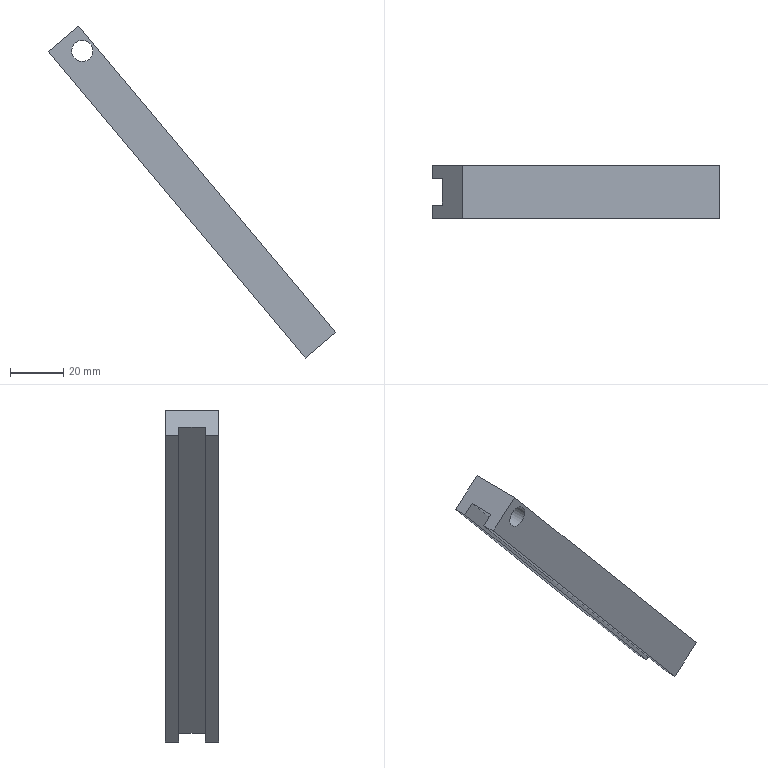Component | NX | MODEL7 | 1 solid | 11 faces | box 107.91 x 20 x 124.55 mm | volume 36495 mm3 | plane 10 | cylinder 1 | commonest cylinder face diameters 8 x1
STEP:
#1=CARTESIAN_POINT('',(0.,0.,0.));
#2=DIRECTION('',(0.,0.,1.));
#3=DIRECTION('',(1.,0.,0.));
#4=AXIS2_PLACEMENT_3D('',#1,#2,#3);
#5=CARTESIAN_POINT('',(827.663,10.431,-119.455));
#6=VERTEX_POINT('',#5);
#7=CARTESIAN_POINT('',(924.081,10.431,-234.362));
#8=VERTEX_POINT('',#7);
#9=CARTESIAN_POINT('',(827.663,10.431,-119.455));
#10=DIRECTION('',(0.6428,0.,-0.766));
#11=VECTOR('',#10,1.);
#12=LINE('',#9,#11);
#13=CARTESIAN_POINT('',(827.663,-4.569,-119.455));
#14=DIRECTION('',(0.766,0.,0.6428));
#15=DIRECTION('',(0.,-1.,0.));
#16=AXIS2_PLACEMENT_3D('',#13,#14,#15);
#17=PLANE('',#16);
#18=CARTESIAN_POINT('',(-15.,0.));
#19=DIRECTION('',(0.,1.));
#20=VECTOR('',#19,1.);
#21=LINE('',#18,#20);
#22=(GEOMETRIC_REPRESENTATION_CONTEXT(2)PARAMETRIC_REPRESENTATION_CONTEXT()REPRESENTATION_CONTEXT('',''));
#23=DEFINITIONAL_REPRESENTATION('',(#21),#22);
#24=PCURVE('',#17,#23);
#25=CARTESIAN_POINT('',(831.493,10.431,-116.241));
#26=DIRECTION('',(0.,1.,0.));
#27=DIRECTION('',(-0.6428,0.,0.766));
#28=AXIS2_PLACEMENT_3D('',#25,#26,#27);
#29=PLANE('',#28);
#30=CARTESIAN_POINT('',(0.,-5.));
#31=DIRECTION('',(-1.,0.));
#32=VECTOR('',#31,1.);
#33=LINE('',#30,#32);
#34=(GEOMETRIC_REPRESENTATION_CONTEXT(2)PARAMETRIC_REPRESENTATION_CONTEXT()REPRESENTATION_CONTEXT('',''));
#35=DEFINITIONAL_REPRESENTATION('',(#33),#34);
#36=PCURVE('',#29,#35);
#37=SURFACE_CURVE('',#12,(#24,#36),.PCURVE_S1.);
#38=EDGE_CURVE('',#6,#8,#37,.T.);
#39=ORIENTED_EDGE('',*,*,#38,.F.);
#40=CARTESIAN_POINT('',(827.663,15.431,-119.455));
#41=VERTEX_POINT('',#40);
#42=CARTESIAN_POINT('',(827.663,-4.569,-119.455));
#43=DIRECTION('',(0.,1.,0.));
#44=VECTOR('',#43,1.);
#45=LINE('',#42,#44);
#46=CARTESIAN_POINT('',(0.,0.));
#47=DIRECTION('',(-1.,0.));
#48=VECTOR('',#47,1.);
#49=LINE('',#46,#48);
#50=(GEOMETRIC_REPRESENTATION_CONTEXT(2)PARAMETRIC_REPRESENTATION_CONTEXT()REPRESENTATION_CONTEXT('',''));
#51=DEFINITIONAL_REPRESENTATION('',(#49),#50);
#52=PCURVE('',#17,#51);
#53=CARTESIAN_POINT('',(839.154,-4.569,-109.813));
#54=DIRECTION('',(0.6428,0.,-0.766));
#55=DIRECTION('',(0.,1.,0.));
#56=AXIS2_PLACEMENT_3D('',#53,#54,#55);
#57=PLANE('',#56);
#58=CARTESIAN_POINT('',(0.,-15.));
#59=DIRECTION('',(1.,0.));
#60=VECTOR('',#59,1.);
#61=LINE('',#58,#60);
#62=(GEOMETRIC_REPRESENTATION_CONTEXT(2)PARAMETRIC_REPRESENTATION_CONTEXT()REPRESENTATION_CONTEXT('',''));
#63=DEFINITIONAL_REPRESENTATION('',(#61),#62);
#64=PCURVE('',#57,#63);
#65=SURFACE_CURVE('',#45,(#52,#64),.PCURVE_S1.);
#66=EDGE_CURVE('',#6,#41,#65,.T.);
#67=ORIENTED_EDGE('',*,*,#66,.T.);
#68=CARTESIAN_POINT('',(924.081,15.431,-234.362));
#69=VERTEX_POINT('',#68);
#70=CARTESIAN_POINT('',(827.663,15.431,-119.455));
#71=DIRECTION('',(0.6428,0.,-0.766));
#72=VECTOR('',#71,1.);
#73=LINE('',#70,#72);
#74=CARTESIAN_POINT('',(-20.,0.));
#75=DIRECTION('',(0.,1.));
#76=VECTOR('',#75,1.);
#77=LINE('',#74,#76);
#78=(GEOMETRIC_REPRESENTATION_CONTEXT(2)PARAMETRIC_REPRESENTATION_CONTEXT()REPRESENTATION_CONTEXT('',''));
#79=DEFINITIONAL_REPRESENTATION('',(#77),#78);
#80=PCURVE('',#17,#79);
#81=CARTESIAN_POINT('',(827.663,15.431,-119.455));
#82=DIRECTION('',(0.,-1.,0.));
#83=DIRECTION('',(0.6428,0.,-0.766));
#84=AXIS2_PLACEMENT_3D('',#81,#82,#83);
#85=PLANE('',#84);
#86=CARTESIAN_POINT('',(0.,0.));
#87=DIRECTION('',(1.,0.));
#88=VECTOR('',#87,1.);
#89=LINE('',#86,#88);
#90=(GEOMETRIC_REPRESENTATION_CONTEXT(2)PARAMETRIC_REPRESENTATION_CONTEXT()REPRESENTATION_CONTEXT('',''));
#91=DEFINITIONAL_REPRESENTATION('',(#89),#90);
#92=PCURVE('',#85,#91);
#93=SURFACE_CURVE('',#73,(#80,#92),.PCURVE_S1.);
#94=EDGE_CURVE('',#41,#69,#93,.T.);
#95=ORIENTED_EDGE('',*,*,#94,.T.);
#96=CARTESIAN_POINT('',(924.081,-4.569,-234.362));
#97=DIRECTION('',(0.,1.,0.));
#98=VECTOR('',#97,1.);
#99=LINE('',#96,#98);
#100=CARTESIAN_POINT('',(0.,150.));
#101=DIRECTION('',(-1.,0.));
#102=VECTOR('',#101,1.);
#103=LINE('',#100,#102);
#104=(GEOMETRIC_REPRESENTATION_CONTEXT(2)PARAMETRIC_REPRESENTATION_CONTEXT()REPRESENTATION_CONTEXT('',''));
#105=DEFINITIONAL_REPRESENTATION('',(#103),#104);
#106=PCURVE('',#17,#105);
#107=CARTESIAN_POINT('',(924.081,-4.569,-234.362));
#108=DIRECTION('',(-0.6428,0.,0.766));
#109=DIRECTION('',(0.,-1.,0.));
#110=AXIS2_PLACEMENT_3D('',#107,#108,#109);
#111=PLANE('',#110);
#112=CARTESIAN_POINT('',(0.,0.));
#113=DIRECTION('',(-1.,0.));
#114=VECTOR('',#113,1.);
#115=LINE('',#112,#114);
#116=(GEOMETRIC_REPRESENTATION_CONTEXT(2)PARAMETRIC_REPRESENTATION_CONTEXT()REPRESENTATION_CONTEXT('',''));
#117=DEFINITIONAL_REPRESENTATION('',(#115),#116);
#118=PCURVE('',#111,#117);
#119=SURFACE_CURVE('',#99,(#106,#118),.PCURVE_S1.);
#120=EDGE_CURVE('',#8,#69,#119,.T.);
#121=ORIENTED_EDGE('',*,*,#120,.F.);
#122=EDGE_LOOP('',(#39,#67,#95,#121));
#123=FACE_BOUND('',#122,.T.);
#124=ADVANCED_FACE('',(#123),#17,.F.);
#125=CARTESIAN_POINT('',(924.081,0.4306,-234.362));
#126=VERTEX_POINT('',#125);
#127=CARTESIAN_POINT('',(827.663,0.4306,-119.455));
#128=VERTEX_POINT('',#127);
#129=CARTESIAN_POINT('',(924.081,0.4306,-234.362));
#130=DIRECTION('',(-0.6428,0.,0.766));
#131=VECTOR('',#130,1.);
#132=LINE('',#129,#131);
#133=CARTESIAN_POINT('',(827.663,-4.569,-119.455));
#134=DIRECTION('',(0.766,0.,0.6428));
#135=DIRECTION('',(0.,-1.,0.));
#136=AXIS2_PLACEMENT_3D('',#133,#134,#135);
#137=PLANE('',#136);
#138=CARTESIAN_POINT('',(-5.,150.));
#139=DIRECTION('',(0.,-1.));
#140=VECTOR('',#139,1.);
#141=LINE('',#138,#140);
#142=(GEOMETRIC_REPRESENTATION_CONTEXT(2)PARAMETRIC_REPRESENTATION_CONTEXT()REPRESENTATION_CONTEXT('',''));
#143=DEFINITIONAL_REPRESENTATION('',(#141),#142);
#144=PCURVE('',#137,#143);
#145=CARTESIAN_POINT('',(927.911,0.4306,-231.148));
#146=DIRECTION('',(0.,-1.,0.));
#147=DIRECTION('',(0.6428,0.,-0.766));
#148=AXIS2_PLACEMENT_3D('',#145,#146,#147);
#149=PLANE('',#148);
#150=CARTESIAN_POINT('',(0.,-5.));
#151=DIRECTION('',(-1.,0.));
#152=VECTOR('',#151,1.);
#153=LINE('',#150,#152);
#154=(GEOMETRIC_REPRESENTATION_CONTEXT(2)PARAMETRIC_REPRESENTATION_CONTEXT()REPRESENTATION_CONTEXT('',''));
#155=DEFINITIONAL_REPRESENTATION('',(#153),#154);
#156=PCURVE('',#149,#155);
#157=SURFACE_CURVE('',#132,(#144,#156),.PCURVE_S1.);
#158=EDGE_CURVE('',#126,#128,#157,.T.);
#159=ORIENTED_EDGE('',*,*,#158,.F.);
#160=CARTESIAN_POINT('',(924.081,-4.569,-234.362));
#161=VERTEX_POINT('',#160);
#162=CARTESIAN_POINT('',(924.081,-4.569,-234.362));
#163=DIRECTION('',(0.,1.,0.));
#164=VECTOR('',#163,1.);
#165=LINE('',#162,#164);
#166=CARTESIAN_POINT('',(0.,150.));
#167=DIRECTION('',(-1.,0.));
#168=VECTOR('',#167,1.);
#169=LINE('',#166,#168);
#170=(GEOMETRIC_REPRESENTATION_CONTEXT(2)PARAMETRIC_REPRESENTATION_CONTEXT()REPRESENTATION_CONTEXT('',''));
#171=DEFINITIONAL_REPRESENTATION('',(#169),#170);
#172=PCURVE('',#137,#171);
#173=CARTESIAN_POINT('',(0.,0.));
#174=DIRECTION('',(-1.,0.));
#175=VECTOR('',#174,1.);
#176=LINE('',#173,#175);
#177=(GEOMETRIC_REPRESENTATION_CONTEXT(2)PARAMETRIC_REPRESENTATION_CONTEXT()REPRESENTATION_CONTEXT('',''));
#178=DEFINITIONAL_REPRESENTATION('',(#176),#177);
#179=PCURVE('',#111,#178);
#180=SURFACE_CURVE('',#165,(#172,#179),.PCURVE_S1.);
#181=EDGE_CURVE('',#161,#126,#180,.T.);
#182=ORIENTED_EDGE('',*,*,#181,.F.);
#183=CARTESIAN_POINT('',(827.663,-4.569,-119.455));
#184=VERTEX_POINT('',#183);
#185=CARTESIAN_POINT('',(827.663,-4.569,-119.455));
#186=DIRECTION('',(0.6428,0.,-0.766));
#187=VECTOR('',#186,1.);
#188=LINE('',#185,#187);
#189=CARTESIAN_POINT('',(0.,0.));
#190=DIRECTION('',(0.,1.));
#191=VECTOR('',#190,1.);
#192=LINE('',#189,#191);
#193=(GEOMETRIC_REPRESENTATION_CONTEXT(2)PARAMETRIC_REPRESENTATION_CONTEXT()REPRESENTATION_CONTEXT('',''));
#194=DEFINITIONAL_REPRESENTATION('',(#192),#193);
#195=PCURVE('',#137,#194);
#196=CARTESIAN_POINT('',(827.663,-4.569,-119.455));
#197=DIRECTION('',(0.,-1.,0.));
#198=DIRECTION('',(0.6428,0.,-0.766));
#199=AXIS2_PLACEMENT_3D('',#196,#197,#198);
#200=PLANE('',#199);
#201=CARTESIAN_POINT('',(0.,0.));
#202=DIRECTION('',(1.,0.));
#203=VECTOR('',#202,1.);
#204=LINE('',#201,#203);
#205=(GEOMETRIC_REPRESENTATION_CONTEXT(2)PARAMETRIC_REPRESENTATION_CONTEXT()REPRESENTATION_CONTEXT('',''));
#206=DEFINITIONAL_REPRESENTATION('',(#204),#205);
#207=PCURVE('',#200,#206);
#208=SURFACE_CURVE('',#188,(#195,#207),.PCURVE_S1.);
#209=EDGE_CURVE('',#184,#161,#208,.T.);
#210=ORIENTED_EDGE('',*,*,#209,.F.);
#211=CARTESIAN_POINT('',(827.663,-4.569,-119.455));
#212=DIRECTION('',(0.,1.,0.));
#213=VECTOR('',#212,1.);
#214=LINE('',#211,#213);
#215=CARTESIAN_POINT('',(0.,0.));
#216=DIRECTION('',(-1.,0.));
#217=VECTOR('',#216,1.);
#218=LINE('',#215,#217);
#219=(GEOMETRIC_REPRESENTATION_CONTEXT(2)PARAMETRIC_REPRESENTATION_CONTEXT()REPRESENTATION_CONTEXT('',''));
#220=DEFINITIONAL_REPRESENTATION('',(#218),#219);
#221=PCURVE('',#137,#220);
#222=CARTESIAN_POINT('',(0.,-15.));
#223=DIRECTION('',(1.,0.));
#224=VECTOR('',#223,1.);
#225=LINE('',#222,#224);
#226=(GEOMETRIC_REPRESENTATION_CONTEXT(2)PARAMETRIC_REPRESENTATION_CONTEXT()REPRESENTATION_CONTEXT('',''));
#227=DEFINITIONAL_REPRESENTATION('',(#225),#226);
#228=PCURVE('',#57,#227);
#229=SURFACE_CURVE('',#214,(#221,#228),.PCURVE_S1.);
#230=EDGE_CURVE('',#184,#128,#229,.T.);
#231=ORIENTED_EDGE('',*,*,#230,.T.);
#232=EDGE_LOOP('',(#159,#182,#210,#231));
#233=FACE_BOUND('',#232,.T.);
#234=ADVANCED_FACE('',(#233),#137,.F.);
#235=CARTESIAN_POINT('',(831.493,0.4306,-116.241));
#236=VERTEX_POINT('',#235);
#237=CARTESIAN_POINT('',(831.493,10.431,-116.241));
#238=VERTEX_POINT('',#237);
#239=CARTESIAN_POINT('',(831.493,0.4306,-116.241));
#240=DIRECTION('',(0.,1.,0.));
#241=VECTOR('',#240,1.);
#242=LINE('',#239,#241);
#243=CARTESIAN_POINT('',(5.,-10.));
#244=DIRECTION('',(1.,0.));
#245=VECTOR('',#244,1.);
#246=LINE('',#243,#245);
#247=(GEOMETRIC_REPRESENTATION_CONTEXT(2)PARAMETRIC_REPRESENTATION_CONTEXT()REPRESENTATION_CONTEXT('',''));
#248=DEFINITIONAL_REPRESENTATION('',(#246),#247);
#249=PCURVE('',#57,#248);
#250=CARTESIAN_POINT('',(831.493,15.431,-116.241));
#251=DIRECTION('',(-0.766,0.,-0.6428));
#252=DIRECTION('',(0.,1.,0.));
#253=AXIS2_PLACEMENT_3D('',#250,#251,#252);
#254=PLANE('',#253);
#255=CARTESIAN_POINT('',(-15.,0.));
#256=DIRECTION('',(1.,0.));
#257=VECTOR('',#256,1.);
#258=LINE('',#255,#257);
#259=(GEOMETRIC_REPRESENTATION_CONTEXT(2)PARAMETRIC_REPRESENTATION_CONTEXT()REPRESENTATION_CONTEXT('',''));
#260=DEFINITIONAL_REPRESENTATION('',(#258),#259);
#261=PCURVE('',#254,#260);
#262=SURFACE_CURVE('',#242,(#249,#261),.PCURVE_S1.);
#263=EDGE_CURVE('',#236,#238,#262,.T.);
#264=ORIENTED_EDGE('',*,*,#263,.F.);
#265=CARTESIAN_POINT('',(831.493,0.4306,-116.241));
#266=DIRECTION('',(-0.766,0.,-0.6428));
#267=VECTOR('',#266,1.);
#268=LINE('',#265,#267);
#269=CARTESIAN_POINT('',(5.,-10.));
#270=DIRECTION('',(0.,-1.));
#271=VECTOR('',#270,1.);
#272=LINE('',#269,#271);
#273=(GEOMETRIC_REPRESENTATION_CONTEXT(2)PARAMETRIC_REPRESENTATION_CONTEXT()REPRESENTATION_CONTEXT('',''));
#274=DEFINITIONAL_REPRESENTATION('',(#272),#273);
#275=PCURVE('',#57,#274);
#276=CARTESIAN_POINT('',(-150.,-0.));
#277=DIRECTION('',(-0.,-1.));
#278=VECTOR('',#277,1.);
#279=LINE('',#276,#278);
#280=(GEOMETRIC_REPRESENTATION_CONTEXT(2)PARAMETRIC_REPRESENTATION_CONTEXT()REPRESENTATION_CONTEXT('',''));
#281=DEFINITIONAL_REPRESENTATION('',(#279),#280);
#282=PCURVE('',#149,#281);
#283=SURFACE_CURVE('',#268,(#275,#282),.PCURVE_S1.);
#284=EDGE_CURVE('',#236,#128,#283,.T.);
#285=ORIENTED_EDGE('',*,*,#284,.T.);
#286=ORIENTED_EDGE('',*,*,#230,.F.);
#287=CARTESIAN_POINT('',(839.154,-4.569,-109.813));
#288=VERTEX_POINT('',#287);
#289=CARTESIAN_POINT('',(839.154,-4.569,-109.813));
#290=DIRECTION('',(-0.766,0.,-0.6428));
#291=VECTOR('',#290,1.);
#292=LINE('',#289,#291);
#293=CARTESIAN_POINT('',(0.,0.));
#294=DIRECTION('',(0.,-1.));
#295=VECTOR('',#294,1.);
#296=LINE('',#293,#295);
#297=(GEOMETRIC_REPRESENTATION_CONTEXT(2)PARAMETRIC_REPRESENTATION_CONTEXT()REPRESENTATION_CONTEXT('',''));
#298=DEFINITIONAL_REPRESENTATION('',(#296),#297);
#299=PCURVE('',#57,#298);
#300=CARTESIAN_POINT('',(-0.,15.));
#301=DIRECTION('',(0.,-1.));
#302=VECTOR('',#301,1.);
#303=LINE('',#300,#302);
#304=(GEOMETRIC_REPRESENTATION_CONTEXT(2)PARAMETRIC_REPRESENTATION_CONTEXT()REPRESENTATION_CONTEXT('',''));
#305=DEFINITIONAL_REPRESENTATION('',(#303),#304);
#306=PCURVE('',#200,#305);
#307=SURFACE_CURVE('',#292,(#299,#306),.PCURVE_S1.);
#308=EDGE_CURVE('',#288,#184,#307,.T.);
#309=ORIENTED_EDGE('',*,*,#308,.F.);
#310=CARTESIAN_POINT('',(839.154,15.431,-109.813));
#311=VERTEX_POINT('',#310);
#312=CARTESIAN_POINT('',(839.154,-4.569,-109.813));
#313=DIRECTION('',(0.,1.,0.));
#314=VECTOR('',#313,1.);
#315=LINE('',#312,#314);
#316=CARTESIAN_POINT('',(0.,0.));
#317=DIRECTION('',(1.,0.));
#318=VECTOR('',#317,1.);
#319=LINE('',#316,#318);
#320=(GEOMETRIC_REPRESENTATION_CONTEXT(2)PARAMETRIC_REPRESENTATION_CONTEXT()REPRESENTATION_CONTEXT('',''));
#321=DEFINITIONAL_REPRESENTATION('',(#319),#320);
#322=PCURVE('',#57,#321);
#323=CARTESIAN_POINT('',(935.572,-4.569,-224.72));
#324=DIRECTION('',(-0.766,0.,-0.6428));
#325=DIRECTION('',(0.,1.,0.));
#326=AXIS2_PLACEMENT_3D('',#323,#324,#325);
#327=PLANE('',#326);
#328=CARTESIAN_POINT('',(0.,-150.));
#329=DIRECTION('',(1.,0.));
#330=VECTOR('',#329,1.);
#331=LINE('',#328,#330);
#332=(GEOMETRIC_REPRESENTATION_CONTEXT(2)PARAMETRIC_REPRESENTATION_CONTEXT()REPRESENTATION_CONTEXT('',''));
#333=DEFINITIONAL_REPRESENTATION('',(#331),#332);
#334=PCURVE('',#327,#333);
#335=SURFACE_CURVE('',#315,(#322,#334),.PCURVE_S1.);
#336=EDGE_CURVE('',#288,#311,#335,.T.);
#337=ORIENTED_EDGE('',*,*,#336,.T.);
#338=CARTESIAN_POINT('',(839.154,15.431,-109.813));
#339=DIRECTION('',(-0.766,0.,-0.6428));
#340=VECTOR('',#339,1.);
#341=LINE('',#338,#340);
#342=CARTESIAN_POINT('',(20.,0.));
#343=DIRECTION('',(0.,-1.));
#344=VECTOR('',#343,1.);
#345=LINE('',#342,#344);
#346=(GEOMETRIC_REPRESENTATION_CONTEXT(2)PARAMETRIC_REPRESENTATION_CONTEXT()REPRESENTATION_CONTEXT('',''));
#347=DEFINITIONAL_REPRESENTATION('',(#345),#346);
#348=PCURVE('',#57,#347);
#349=CARTESIAN_POINT('',(-0.,15.));
#350=DIRECTION('',(0.,-1.));
#351=VECTOR('',#350,1.);
#352=LINE('',#349,#351);
#353=(GEOMETRIC_REPRESENTATION_CONTEXT(2)PARAMETRIC_REPRESENTATION_CONTEXT()REPRESENTATION_CONTEXT('',''));
#354=DEFINITIONAL_REPRESENTATION('',(#352),#353);
#355=PCURVE('',#85,#354);
#356=SURFACE_CURVE('',#341,(#348,#355),.PCURVE_S1.);
#357=EDGE_CURVE('',#311,#41,#356,.T.);
#358=ORIENTED_EDGE('',*,*,#357,.T.);
#359=ORIENTED_EDGE('',*,*,#66,.F.);
#360=CARTESIAN_POINT('',(831.493,10.431,-116.241));
#361=DIRECTION('',(-0.766,0.,-0.6428));
#362=VECTOR('',#361,1.);
#363=LINE('',#360,#362);
#364=CARTESIAN_POINT('',(15.,-10.));
#365=DIRECTION('',(0.,-1.));
#366=VECTOR('',#365,1.);
#367=LINE('',#364,#366);
#368=(GEOMETRIC_REPRESENTATION_CONTEXT(2)PARAMETRIC_REPRESENTATION_CONTEXT()REPRESENTATION_CONTEXT('',''));
#369=DEFINITIONAL_REPRESENTATION('',(#367),#368);
#370=PCURVE('',#57,#369);
#371=CARTESIAN_POINT('',(0.,0.));
#372=DIRECTION('',(0.,-1.));
#373=VECTOR('',#372,1.);
#374=LINE('',#371,#373);
#375=(GEOMETRIC_REPRESENTATION_CONTEXT(2)PARAMETRIC_REPRESENTATION_CONTEXT()REPRESENTATION_CONTEXT('',''));
#376=DEFINITIONAL_REPRESENTATION('',(#374),#375);
#377=PCURVE('',#29,#376);
#378=SURFACE_CURVE('',#363,(#370,#377),.PCURVE_S1.);
#379=EDGE_CURVE('',#238,#6,#378,.T.);
#380=ORIENTED_EDGE('',*,*,#379,.F.);
#381=EDGE_LOOP('',(#264,#285,#286,#309,#337,#358,#359,#380));
#382=FACE_BOUND('',#381,.T.);
#383=ADVANCED_FACE('',(#382),#57,.F.);
#384=CARTESIAN_POINT('',(927.911,10.431,-231.148));
#385=VERTEX_POINT('',#384);
#386=CARTESIAN_POINT('',(927.911,0.4306,-231.148));
#387=VERTEX_POINT('',#386);
#388=CARTESIAN_POINT('',(927.911,10.431,-231.148));
#389=DIRECTION('',(0.,-1.,0.));
#390=VECTOR('',#389,1.);
#391=LINE('',#388,#390);
#392=CARTESIAN_POINT('',(-15.,5.));
#393=DIRECTION('',(1.,0.));
#394=VECTOR('',#393,1.);
#395=LINE('',#392,#394);
#396=(GEOMETRIC_REPRESENTATION_CONTEXT(2)PARAMETRIC_REPRESENTATION_CONTEXT()REPRESENTATION_CONTEXT('',''));
#397=DEFINITIONAL_REPRESENTATION('',(#395),#396);
#398=PCURVE('',#111,#397);
#399=CARTESIAN_POINT('',(-5.,150.));
#400=DIRECTION('',(-1.,0.));
#401=VECTOR('',#400,1.);
#402=LINE('',#399,#401);
#403=(GEOMETRIC_REPRESENTATION_CONTEXT(2)PARAMETRIC_REPRESENTATION_CONTEXT()REPRESENTATION_CONTEXT('',''));
#404=DEFINITIONAL_REPRESENTATION('',(#402),#403);
#405=PCURVE('',#254,#404);
#406=SURFACE_CURVE('',#391,(#398,#405),.PCURVE_S1.);
#407=EDGE_CURVE('',#385,#387,#406,.T.);
#408=ORIENTED_EDGE('',*,*,#407,.F.);
#409=CARTESIAN_POINT('',(927.911,10.431,-231.148));
#410=DIRECTION('',(-0.766,0.,-0.6428));
#411=VECTOR('',#410,1.);
#412=LINE('',#409,#411);
#413=CARTESIAN_POINT('',(-15.,5.));
#414=DIRECTION('',(0.,-1.));
#415=VECTOR('',#414,1.);
#416=LINE('',#413,#415);
#417=(GEOMETRIC_REPRESENTATION_CONTEXT(2)PARAMETRIC_REPRESENTATION_CONTEXT()REPRESENTATION_CONTEXT('',''));
#418=DEFINITIONAL_REPRESENTATION('',(#416),#417);
#419=PCURVE('',#111,#418);
#420=CARTESIAN_POINT('',(-150.,0.));
#421=DIRECTION('',(0.,-1.));
#422=VECTOR('',#421,1.);
#423=LINE('',#420,#422);
#424=(GEOMETRIC_REPRESENTATION_CONTEXT(2)PARAMETRIC_REPRESENTATION_CONTEXT()REPRESENTATION_CONTEXT('',''));
#425=DEFINITIONAL_REPRESENTATION('',(#423),#424);
#426=PCURVE('',#29,#425);
#427=SURFACE_CURVE('',#412,(#419,#426),.PCURVE_S1.);
#428=EDGE_CURVE('',#385,#8,#427,.T.);
#429=ORIENTED_EDGE('',*,*,#428,.T.);
#430=ORIENTED_EDGE('',*,*,#120,.T.);
#431=CARTESIAN_POINT('',(935.572,15.431,-224.72));
#432=VERTEX_POINT('',#431);
#433=CARTESIAN_POINT('',(924.081,15.431,-234.362));
#434=DIRECTION('',(0.766,0.,0.6428));
#435=VECTOR('',#434,1.);
#436=LINE('',#433,#435);
#437=CARTESIAN_POINT('',(-20.,0.));
#438=DIRECTION('',(0.,1.));
#439=VECTOR('',#438,1.);
#440=LINE('',#437,#439);
#441=(GEOMETRIC_REPRESENTATION_CONTEXT(2)PARAMETRIC_REPRESENTATION_CONTEXT()REPRESENTATION_CONTEXT('',''));
#442=DEFINITIONAL_REPRESENTATION('',(#440),#441);
#443=PCURVE('',#111,#442);
#444=CARTESIAN_POINT('',(150.,0.));
#445=DIRECTION('',(0.,1.));
#446=VECTOR('',#445,1.);
#447=LINE('',#444,#446);
#448=(GEOMETRIC_REPRESENTATION_CONTEXT(2)PARAMETRIC_REPRESENTATION_CONTEXT()REPRESENTATION_CONTEXT('',''));
#449=DEFINITIONAL_REPRESENTATION('',(#447),#448);
#450=PCURVE('',#85,#449);
#451=SURFACE_CURVE('',#436,(#443,#450),.PCURVE_S1.);
#452=EDGE_CURVE('',#69,#432,#451,.T.);
#453=ORIENTED_EDGE('',*,*,#452,.T.);
#454=CARTESIAN_POINT('',(935.572,-4.569,-224.72));
#455=VERTEX_POINT('',#454);
#456=CARTESIAN_POINT('',(935.572,-4.569,-224.72));
#457=DIRECTION('',(0.,1.,0.));
#458=VECTOR('',#457,1.);
#459=LINE('',#456,#458);
#460=CARTESIAN_POINT('',(0.,15.));
#461=DIRECTION('',(-1.,0.));
#462=VECTOR('',#461,1.);
#463=LINE('',#460,#462);
#464=(GEOMETRIC_REPRESENTATION_CONTEXT(2)PARAMETRIC_REPRESENTATION_CONTEXT()REPRESENTATION_CONTEXT('',''));
#465=DEFINITIONAL_REPRESENTATION('',(#463),#464);
#466=PCURVE('',#111,#465);
#467=CARTESIAN_POINT('',(0.,0.));
#468=DIRECTION('',(1.,0.));
#469=VECTOR('',#468,1.);
#470=LINE('',#467,#469);
#471=(GEOMETRIC_REPRESENTATION_CONTEXT(2)PARAMETRIC_REPRESENTATION_CONTEXT()REPRESENTATION_CONTEXT('',''));
#472=DEFINITIONAL_REPRESENTATION('',(#470),#471);
#473=PCURVE('',#327,#472);
#474=SURFACE_CURVE('',#459,(#466,#473),.PCURVE_S1.);
#475=EDGE_CURVE('',#455,#432,#474,.T.);
#476=ORIENTED_EDGE('',*,*,#475,.F.);
#477=CARTESIAN_POINT('',(924.081,-4.569,-234.362));
#478=DIRECTION('',(0.766,0.,0.6428));
#479=VECTOR('',#478,1.);
#480=LINE('',#477,#479);
#481=CARTESIAN_POINT('',(0.,0.));
#482=DIRECTION('',(0.,1.));
#483=VECTOR('',#482,1.);
#484=LINE('',#481,#483);
#485=(GEOMETRIC_REPRESENTATION_CONTEXT(2)PARAMETRIC_REPRESENTATION_CONTEXT()REPRESENTATION_CONTEXT('',''));
#486=DEFINITIONAL_REPRESENTATION('',(#484),#485);
#487=PCURVE('',#111,#486);
#488=CARTESIAN_POINT('',(150.,0.));
#489=DIRECTION('',(0.,1.));
#490=VECTOR('',#489,1.);
#491=LINE('',#488,#490);
#492=(GEOMETRIC_REPRESENTATION_CONTEXT(2)PARAMETRIC_REPRESENTATION_CONTEXT()REPRESENTATION_CONTEXT('',''));
#493=DEFINITIONAL_REPRESENTATION('',(#491),#492);
#494=PCURVE('',#200,#493);
#495=SURFACE_CURVE('',#480,(#487,#494),.PCURVE_S1.);
#496=EDGE_CURVE('',#161,#455,#495,.T.);
#497=ORIENTED_EDGE('',*,*,#496,.F.);
#498=ORIENTED_EDGE('',*,*,#181,.T.);
#499=CARTESIAN_POINT('',(927.911,0.4306,-231.148));
#500=DIRECTION('',(-0.766,0.,-0.6428));
#501=VECTOR('',#500,1.);
#502=LINE('',#499,#501);
#503=CARTESIAN_POINT('',(-5.,5.));
#504=DIRECTION('',(0.,-1.));
#505=VECTOR('',#504,1.);
#506=LINE('',#503,#505);
#507=(GEOMETRIC_REPRESENTATION_CONTEXT(2)PARAMETRIC_REPRESENTATION_CONTEXT()REPRESENTATION_CONTEXT('',''));
#508=DEFINITIONAL_REPRESENTATION('',(#506),#507);
#509=PCURVE('',#111,#508);
#510=CARTESIAN_POINT('',(0.,0.));
#511=DIRECTION('',(-0.,-1.));
#512=VECTOR('',#511,1.);
#513=LINE('',#510,#512);
#514=(GEOMETRIC_REPRESENTATION_CONTEXT(2)PARAMETRIC_REPRESENTATION_CONTEXT()REPRESENTATION_CONTEXT('',''));
#515=DEFINITIONAL_REPRESENTATION('',(#513),#514);
#516=PCURVE('',#149,#515);
#517=SURFACE_CURVE('',#502,(#509,#516),.PCURVE_S1.);
#518=EDGE_CURVE('',#387,#126,#517,.T.);
#519=ORIENTED_EDGE('',*,*,#518,.F.);
#520=EDGE_LOOP('',(#408,#429,#430,#453,#476,#497,#498,#519));
#521=FACE_BOUND('',#520,.T.);
#522=ADVANCED_FACE('',(#521),#111,.F.);
#523=CARTESIAN_POINT('',(935.572,15.431,-224.72));
#524=DIRECTION('',(-0.6428,0.,0.766));
#525=VECTOR('',#524,1.);
#526=LINE('',#523,#525);
#527=CARTESIAN_POINT('',(20.,0.));
#528=DIRECTION('',(0.,-1.));
#529=VECTOR('',#528,1.);
#530=LINE('',#527,#529);
#531=(GEOMETRIC_REPRESENTATION_CONTEXT(2)PARAMETRIC_REPRESENTATION_CONTEXT()REPRESENTATION_CONTEXT('',''));
#532=DEFINITIONAL_REPRESENTATION('',(#530),#531);
#533=PCURVE('',#327,#532);
#534=CARTESIAN_POINT('',(150.,15.));
#535=DIRECTION('',(-1.,0.));
#536=VECTOR('',#535,1.);
#537=LINE('',#534,#536);
#538=(GEOMETRIC_REPRESENTATION_CONTEXT(2)PARAMETRIC_REPRESENTATION_CONTEXT()REPRESENTATION_CONTEXT('',''));
#539=DEFINITIONAL_REPRESENTATION('',(#537),#538);
#540=PCURVE('',#85,#539);
#541=SURFACE_CURVE('',#526,(#533,#540),.PCURVE_S1.);
#542=EDGE_CURVE('',#432,#311,#541,.T.);
#543=ORIENTED_EDGE('',*,*,#542,.T.);
#544=ORIENTED_EDGE('',*,*,#336,.F.);
#545=CARTESIAN_POINT('',(935.572,-4.569,-224.72));
#546=DIRECTION('',(-0.6428,0.,0.766));
#547=VECTOR('',#546,1.);
#548=LINE('',#545,#547);
#549=CARTESIAN_POINT('',(0.,0.));
#550=DIRECTION('',(0.,-1.));
#551=VECTOR('',#550,1.);
#552=LINE('',#549,#551);
#553=(GEOMETRIC_REPRESENTATION_CONTEXT(2)PARAMETRIC_REPRESENTATION_CONTEXT()REPRESENTATION_CONTEXT('',''));
#554=DEFINITIONAL_REPRESENTATION('',(#552),#553);
#555=PCURVE('',#327,#554);
#556=CARTESIAN_POINT('',(150.,15.));
#557=DIRECTION('',(-1.,0.));
#558=VECTOR('',#557,1.);
#559=LINE('',#556,#558);
#560=(GEOMETRIC_REPRESENTATION_CONTEXT(2)PARAMETRIC_REPRESENTATION_CONTEXT()REPRESENTATION_CONTEXT('',''));
#561=DEFINITIONAL_REPRESENTATION('',(#559),#560);
#562=PCURVE('',#200,#561);
#563=SURFACE_CURVE('',#548,(#555,#562),.PCURVE_S1.);
#564=EDGE_CURVE('',#455,#288,#563,.T.);
#565=ORIENTED_EDGE('',*,*,#564,.F.);
#566=ORIENTED_EDGE('',*,*,#475,.T.);
#567=EDGE_LOOP('',(#543,#544,#565,#566));
#568=FACE_BOUND('',#567,.T.);
#569=ADVANCED_FACE('',(#568),#327,.F.);
#570=CARTESIAN_POINT('',(837.895,-4.569,-116.091));
#571=VERTEX_POINT('',#570);
#572=CARTESIAN_POINT('',(840.466,-4.569,-119.155));
#573=DIRECTION('',(0.,1.,0.));
#574=DIRECTION('',(-0.6428,0.,0.766));
#575=AXIS2_PLACEMENT_3D('',#572,#573,#574);
#576=CIRCLE('',#575,4.);
#577=CARTESIAN_POINT('',(4.,10.));
#578=CARTESIAN_POINT('',(4.,16.928));
#579=CARTESIAN_POINT('',(10.,13.464));
#580=CARTESIAN_POINT('',(16.,10.));
#581=CARTESIAN_POINT('',(10.,6.536));
#582=CARTESIAN_POINT('',(4.,3.072));
#583=CARTESIAN_POINT('',(4.,10.));
#584=(BOUNDED_CURVE()B_SPLINE_CURVE(2,(#577,#578,#579,#580,#581,#582,#583),.UNSPECIFIED.,.T.,.F.)B_SPLINE_CURVE_WITH_KNOTS((1,2,2,2,2,1),(-2.094,0.,2.094,4.189,6.283,8.378),.UNSPECIFIED.)CURVE()GEOMETRIC_REPRESENTATION_ITEM()RATIONAL_B_SPLINE_CURVE((1.,0.5,1.,0.5,1.,0.5,1.))REPRESENTATION_ITEM(''));
#585=(GEOMETRIC_REPRESENTATION_CONTEXT(2)PARAMETRIC_REPRESENTATION_CONTEXT()REPRESENTATION_CONTEXT('',''));
#586=DEFINITIONAL_REPRESENTATION('',(#584),#585);
#587=PCURVE('',#200,#586);
#588=CARTESIAN_POINT('',(840.466,-4.569,-119.155));
#589=DIRECTION('',(0.,1.,0.));
#590=DIRECTION('',(-0.6428,0.,0.766));
#591=AXIS2_PLACEMENT_3D('',#588,#589,#590);
#592=CYLINDRICAL_SURFACE('',#591,4.);
#593=CARTESIAN_POINT('',(0.,0.));
#594=DIRECTION('',(1.,0.));
#595=VECTOR('',#594,1.);
#596=LINE('',#593,#595);
#597=(GEOMETRIC_REPRESENTATION_CONTEXT(2)PARAMETRIC_REPRESENTATION_CONTEXT()REPRESENTATION_CONTEXT('',''));
#598=DEFINITIONAL_REPRESENTATION('',(#596),#597);
#599=PCURVE('',#592,#598);
#600=SURFACE_CURVE('',#576,(#587,#599),.PCURVE_S1.);
#601=EDGE_CURVE('',#571,#571,#600,.T.);
#602=ORIENTED_EDGE('',*,*,#601,.T.);
#603=EDGE_LOOP('',(#602));
#604=FACE_BOUND('',#603,.T.);
#605=ORIENTED_EDGE('',*,*,#308,.T.);
#606=ORIENTED_EDGE('',*,*,#209,.T.);
#607=ORIENTED_EDGE('',*,*,#496,.T.);
#608=ORIENTED_EDGE('',*,*,#564,.T.);
#609=EDGE_LOOP('',(#605,#606,#607,#608));
#610=FACE_BOUND('',#609,.T.);
#611=ADVANCED_FACE('',(#604,#610),#200,.T.);
#612=CARTESIAN_POINT('',(843.037,15.431,-122.22));
#613=VERTEX_POINT('',#612);
#614=CARTESIAN_POINT('',(837.895,15.431,-116.091));
#615=VERTEX_POINT('',#614);
#616=CARTESIAN_POINT('',(840.466,15.431,-119.155));
#617=DIRECTION('',(0.,-1.,0.));
#618=DIRECTION('',(0.6428,0.,-0.766));
#619=AXIS2_PLACEMENT_3D('',#616,#617,#618);
#620=CIRCLE('',#619,4.);
#621=CARTESIAN_POINT('',(8.,10.));
#622=DIRECTION('',(1.,0.));
#623=AXIS2_PLACEMENT_2D('',#621,#622);
#624=CIRCLE('',#623,4.);
#625=(GEOMETRIC_REPRESENTATION_CONTEXT(2)PARAMETRIC_REPRESENTATION_CONTEXT()REPRESENTATION_CONTEXT('',''));
#626=DEFINITIONAL_REPRESENTATION('',(#624),#625);
#627=PCURVE('',#85,#626);
#628=CARTESIAN_POINT('',(3.142,20.));
#629=DIRECTION('',(-1.,0.));
#630=VECTOR('',#629,1.);
#631=LINE('',#628,#630);
#632=(GEOMETRIC_REPRESENTATION_CONTEXT(2)PARAMETRIC_REPRESENTATION_CONTEXT()REPRESENTATION_CONTEXT('',''));
#633=DEFINITIONAL_REPRESENTATION('',(#631),#632);
#634=PCURVE('',#592,#633);
#635=SURFACE_CURVE('',#620,(#627,#634),.PCURVE_S1.);
#636=EDGE_CURVE('',#613,#615,#635,.T.);
#637=ORIENTED_EDGE('',*,*,#636,.T.);
#638=CARTESIAN_POINT('',(840.466,15.431,-119.155));
#639=DIRECTION('',(0.,-1.,0.));
#640=DIRECTION('',(0.6428,0.,-0.766));
#641=AXIS2_PLACEMENT_3D('',#638,#639,#640);
#642=CIRCLE('',#641,4.);
#643=CARTESIAN_POINT('',(8.,10.));
#644=DIRECTION('',(1.,0.));
#645=AXIS2_PLACEMENT_2D('',#643,#644);
#646=CIRCLE('',#645,4.);
#647=(GEOMETRIC_REPRESENTATION_CONTEXT(2)PARAMETRIC_REPRESENTATION_CONTEXT()REPRESENTATION_CONTEXT('',''));
#648=DEFINITIONAL_REPRESENTATION('',(#646),#647);
#649=PCURVE('',#85,#648);
#650=CARTESIAN_POINT('',(9.425,20.));
#651=DIRECTION('',(-1.,0.));
#652=VECTOR('',#651,1.);
#653=LINE('',#650,#652);
#654=(GEOMETRIC_REPRESENTATION_CONTEXT(2)PARAMETRIC_REPRESENTATION_CONTEXT()REPRESENTATION_CONTEXT('',''));
#655=DEFINITIONAL_REPRESENTATION('',(#653),#654);
#656=PCURVE('',#592,#655);
#657=SURFACE_CURVE('',#642,(#649,#656),.PCURVE_S1.);
#658=EDGE_CURVE('',#615,#613,#657,.T.);
#659=ORIENTED_EDGE('',*,*,#658,.T.);
#660=EDGE_LOOP('',(#637,#659));
#661=FACE_BOUND('',#660,.T.);
#662=ORIENTED_EDGE('',*,*,#357,.F.);
#663=ORIENTED_EDGE('',*,*,#542,.F.);
#664=ORIENTED_EDGE('',*,*,#452,.F.);
#665=ORIENTED_EDGE('',*,*,#94,.F.);
#666=EDGE_LOOP('',(#662,#663,#664,#665));
#667=FACE_BOUND('',#666,.T.);
#668=ADVANCED_FACE('',(#661,#667),#85,.F.);
#669=ORIENTED_EDGE('',*,*,#38,.T.);
#670=ORIENTED_EDGE('',*,*,#428,.F.);
#671=CARTESIAN_POINT('',(831.493,10.431,-116.241));
#672=DIRECTION('',(-0.6428,0.,0.766));
#673=VECTOR('',#672,1.);
#674=LINE('',#671,#673);
#675=CARTESIAN_POINT('',(0.,0.));
#676=DIRECTION('',(1.,0.));
#677=VECTOR('',#676,1.);
#678=LINE('',#675,#677);
#679=(GEOMETRIC_REPRESENTATION_CONTEXT(2)PARAMETRIC_REPRESENTATION_CONTEXT()REPRESENTATION_CONTEXT('',''));
#680=DEFINITIONAL_REPRESENTATION('',(#678),#679);
#681=PCURVE('',#29,#680);
#682=CARTESIAN_POINT('',(-5.,0.));
#683=DIRECTION('',(0.,-1.));
#684=VECTOR('',#683,1.);
#685=LINE('',#682,#684);
#686=(GEOMETRIC_REPRESENTATION_CONTEXT(2)PARAMETRIC_REPRESENTATION_CONTEXT()REPRESENTATION_CONTEXT('',''));
#687=DEFINITIONAL_REPRESENTATION('',(#685),#686);
#688=PCURVE('',#254,#687);
#689=SURFACE_CURVE('',#674,(#681,#688),.PCURVE_S1.);
#690=EDGE_CURVE('',#385,#238,#689,.T.);
#691=ORIENTED_EDGE('',*,*,#690,.T.);
#692=ORIENTED_EDGE('',*,*,#379,.T.);
#693=EDGE_LOOP('',(#669,#670,#691,#692));
#694=FACE_BOUND('',#693,.T.);
#695=ADVANCED_FACE('',(#694),#29,.F.);
#696=ORIENTED_EDGE('',*,*,#158,.T.);
#697=ORIENTED_EDGE('',*,*,#284,.F.);
#698=CARTESIAN_POINT('',(927.911,0.4306,-231.148));
#699=DIRECTION('',(0.6428,0.,-0.766));
#700=VECTOR('',#699,1.);
#701=LINE('',#698,#700);
#702=CARTESIAN_POINT('',(0.,0.));
#703=DIRECTION('',(1.,-0.));
#704=VECTOR('',#703,1.);
#705=LINE('',#702,#704);
#706=(GEOMETRIC_REPRESENTATION_CONTEXT(2)PARAMETRIC_REPRESENTATION_CONTEXT()REPRESENTATION_CONTEXT('',''));
#707=DEFINITIONAL_REPRESENTATION('',(#705),#706);
#708=PCURVE('',#149,#707);
#709=CARTESIAN_POINT('',(-15.,150.));
#710=DIRECTION('',(0.,1.));
#711=VECTOR('',#710,1.);
#712=LINE('',#709,#711);
#713=(GEOMETRIC_REPRESENTATION_CONTEXT(2)PARAMETRIC_REPRESENTATION_CONTEXT()REPRESENTATION_CONTEXT('',''));
#714=DEFINITIONAL_REPRESENTATION('',(#712),#713);
#715=PCURVE('',#254,#714);
#716=SURFACE_CURVE('',#701,(#708,#715),.PCURVE_S1.);
#717=EDGE_CURVE('',#236,#387,#716,.T.);
#718=ORIENTED_EDGE('',*,*,#717,.T.);
#719=ORIENTED_EDGE('',*,*,#518,.T.);
#720=EDGE_LOOP('',(#696,#697,#718,#719));
#721=FACE_BOUND('',#720,.T.);
#722=ADVANCED_FACE('',(#721),#149,.F.);
#723=ORIENTED_EDGE('',*,*,#263,.T.);
#724=ORIENTED_EDGE('',*,*,#690,.F.);
#725=ORIENTED_EDGE('',*,*,#407,.T.);
#726=ORIENTED_EDGE('',*,*,#717,.F.);
#727=EDGE_LOOP('',(#723,#724,#725,#726));
#728=FACE_BOUND('',#727,.T.);
#729=ADVANCED_FACE('',(#728),#254,.T.);
#730=ORIENTED_EDGE('',*,*,#601,.T.);
#731=CARTESIAN_POINT('',(837.895,-4.569,-116.091));
#732=CARTESIAN_POINT('',(837.895,15.431,-116.091));
#733=B_SPLINE_CURVE_WITH_KNOTS('',1,(#731,#732),.UNSPECIFIED.,.F.,.F.,(2,2),(0.,20.),.PIECEWISE_BEZIER_KNOTS.);
#734=CARTESIAN_POINT('',(6.283,0.));
#735=DIRECTION('',(0.,1.));
#736=VECTOR('',#735,1.);
#737=LINE('',#734,#736);
#738=(GEOMETRIC_REPRESENTATION_CONTEXT(2)PARAMETRIC_REPRESENTATION_CONTEXT()REPRESENTATION_CONTEXT('',''));
#739=DEFINITIONAL_REPRESENTATION('',(#737),#738);
#740=PCURVE('',#592,#739);
#741=CARTESIAN_POINT('',(0.,0.));
#742=DIRECTION('',(0.,1.));
#743=VECTOR('',#742,1.);
#744=LINE('',#741,#743);
#745=(GEOMETRIC_REPRESENTATION_CONTEXT(2)PARAMETRIC_REPRESENTATION_CONTEXT()REPRESENTATION_CONTEXT('',''));
#746=DEFINITIONAL_REPRESENTATION('',(#744),#745);
#747=PCURVE('',#592,#746);
#748=SEAM_CURVE('',#733,(#740,#747),.PCURVE_S1.);
#749=EDGE_CURVE('',#571,#615,#748,.T.);
#750=ORIENTED_EDGE('',*,*,#749,.T.);
#751=ORIENTED_EDGE('',*,*,#658,.T.);
#752=ORIENTED_EDGE('',*,*,#636,.T.);
#753=ORIENTED_EDGE('',*,*,#749,.F.);
#754=EDGE_LOOP('',(#730,#750,#751,#752,#753));
#755=FACE_BOUND('',#754,.F.);
#756=ADVANCED_FACE('',(#755),#592,.F.);
#757=CLOSED_SHELL('',(#124,#234,#383,#522,#569,#611,#668,#695,#722,#729,#756));
#758=MANIFOLD_SOLID_BREP('',#757);
#759=(LENGTH_UNIT()NAMED_UNIT(*)SI_UNIT(.MILLI.,.METRE.));
#760=UNCERTAINTY_MEASURE_WITH_UNIT(LENGTH_MEASURE(0.000001),#759,'','');
#761=(NAMED_UNIT(*)PLANE_ANGLE_UNIT()SI_UNIT($,.RADIAN.));
#762=(NAMED_UNIT(*)SI_UNIT($,.STERADIAN.)SOLID_ANGLE_UNIT());
#763=(GEOMETRIC_REPRESENTATION_CONTEXT(3)GLOBAL_UNCERTAINTY_ASSIGNED_CONTEXT((#760))GLOBAL_UNIT_ASSIGNED_CONTEXT((#759,#761,#762))REPRESENTATION_CONTEXT('',''));
#764=ADVANCED_BREP_SHAPE_REPRESENTATION('',(#4,#758),#763);